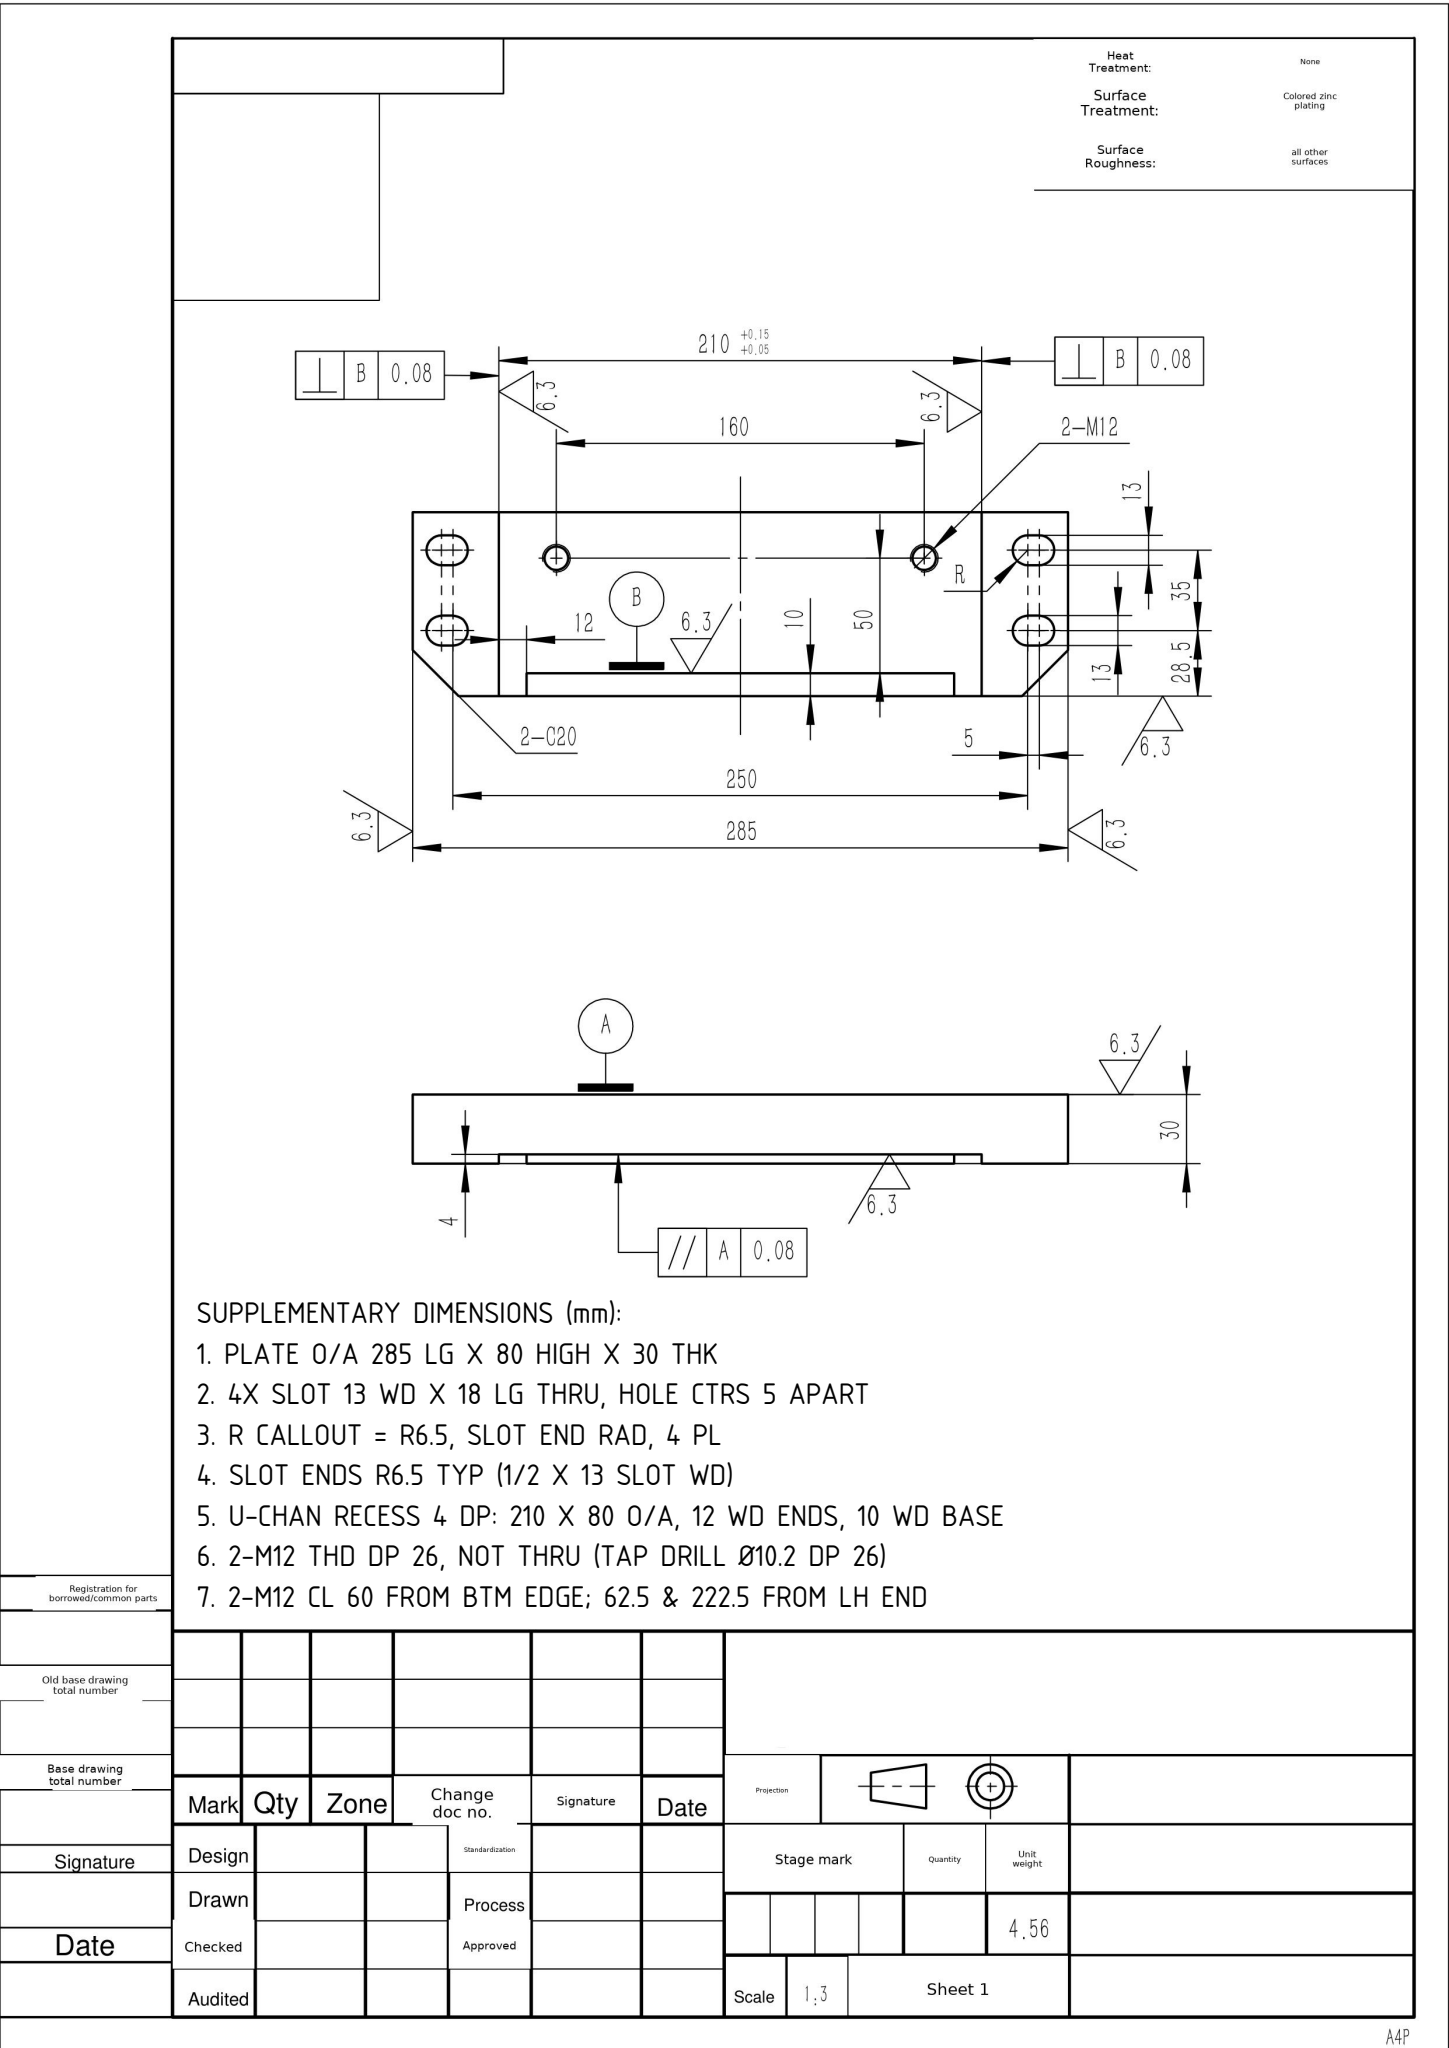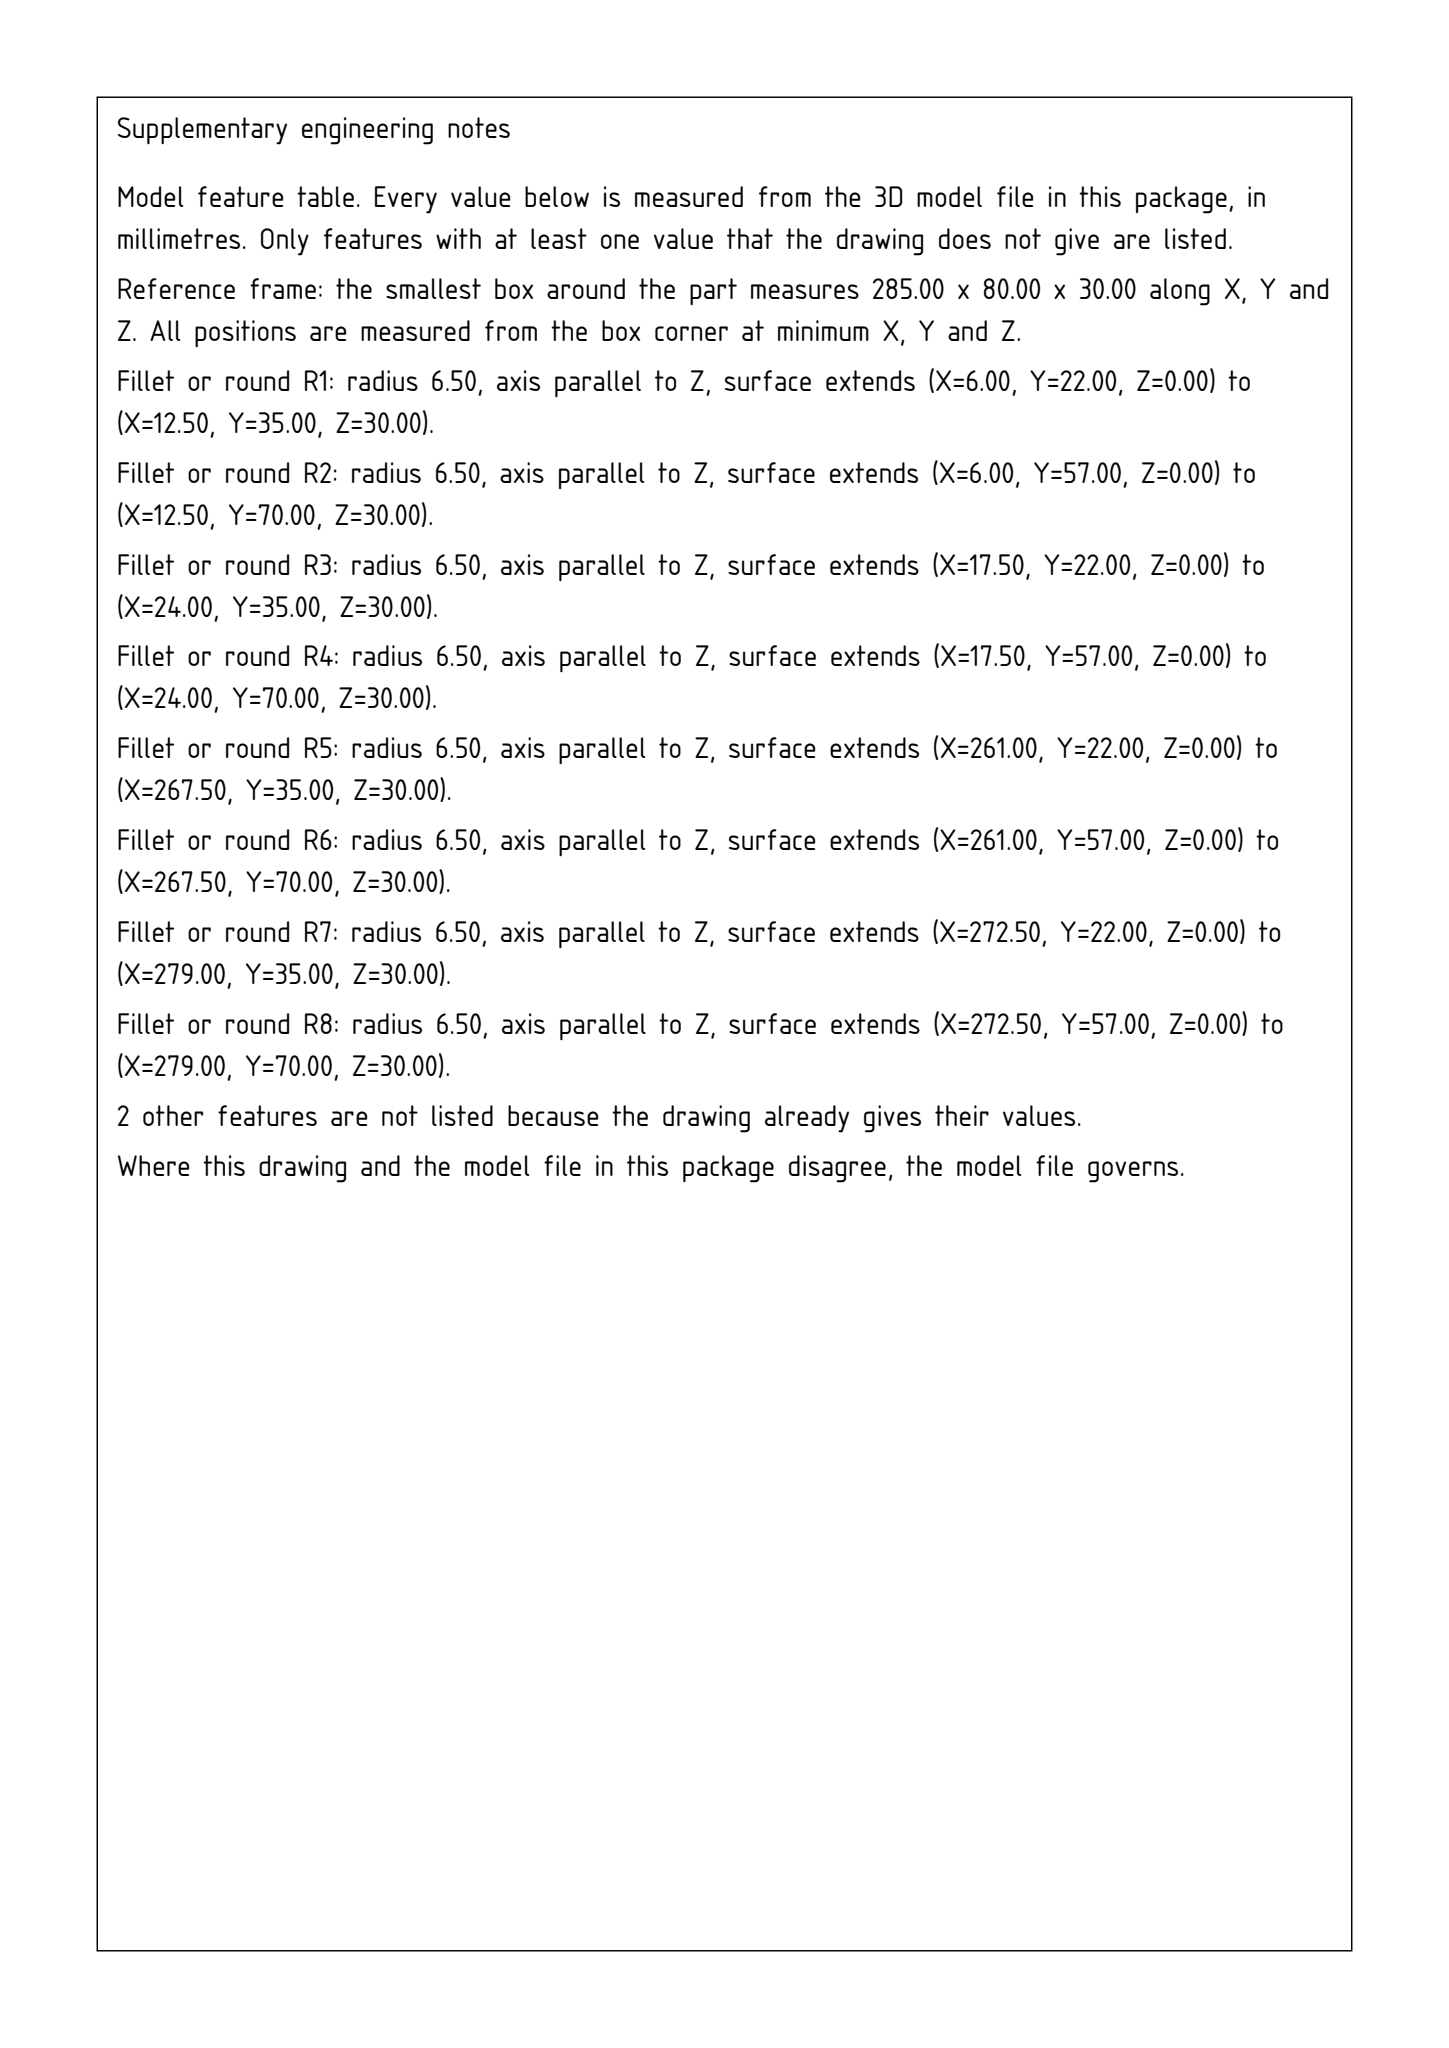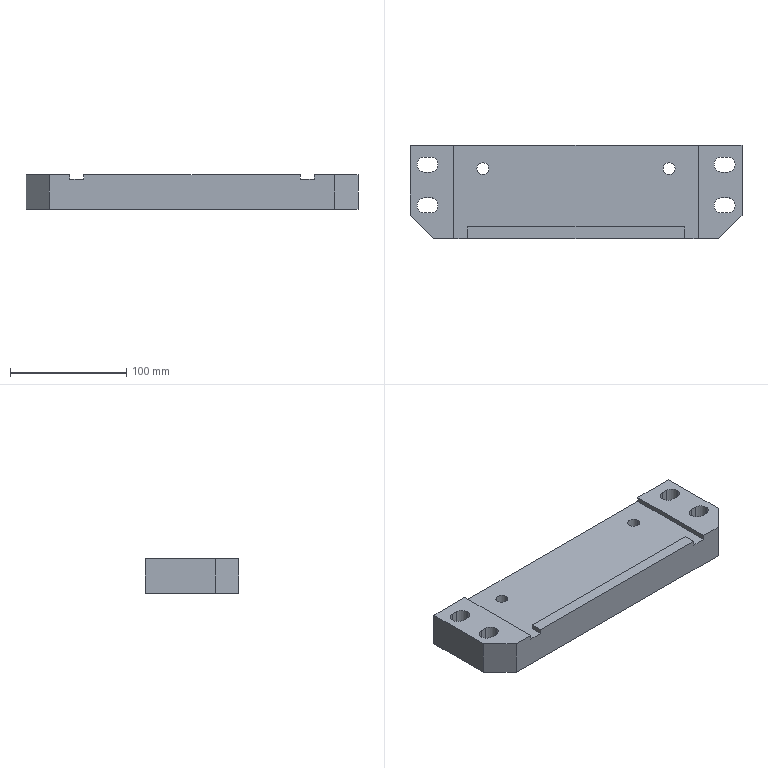Part | SolidWorks | mm | 1 solid | 40 faces | box 285 x 80 x 30 mm | volume 584263 mm3 | plane 24 | cylinder 16 | commonest cylinder face diameters 13 x12 10.2 x4
build123d program:
from build123d import *

# Parameters (mm, degrees)
SKETCH1_W              = 285
SKETCH1_H              = 80
BOSS_EXTRUDE1_DEPTH    = 30
CUT_EXTRUDE1_DEPTH     = 4
CUT_EXTRUDE2_DEPTH     = 152.017
CHAMFER1_SIZE          = 20
M12_TAPPED_HOLE1_D     = 10.2
M12_TAPPED_HOLE1_DEPTH = 29.25
M12_TAPPED_HOLE1_TIP   = 3.064


with BuildPart() as part:
    # Sketch1 → Boss-Extrude1 (new body)
    with BuildSketch(Plane.XY):
        Rectangle(SKETCH1_W, SKETCH1_H)
    extrude(amount=BOSS_EXTRUDE1_DEPTH)

    # Sketch2 → Cut-Extrude1 (cut)
    with BuildSketch(Plane.XY.offset(30)):
        Polygon((-105, 40), (105, 40), (105, -40), (93, -40), (93, -30), (-93, -30), (-93, -40), (-105, -40), align=None)
    extrude(amount=-CUT_EXTRUDE1_DEPTH, mode=Mode.SUBTRACT)

    # Sketch3 → Cut-Extrude2 (cut, through all)
    with BuildSketch(Plane.XY.offset(30)):
        with BuildLine():
            Line((-130, 30), (-125, 30))
            ThreePointArc((-125, 30), (-118.5, 23.5), (-125, 17))
            Line((-125, 17), (-130, 17))
            ThreePointArc((-130, 17), (-136.5, 23.5), (-130, 30))
        make_face()
        with BuildLine():
            Line((130, 30), (125, 30))
            ThreePointArc((125, 30), (118.5, 23.5), (125, 17))
            Line((125, 17), (130, 17))
            ThreePointArc((130, 17), (136.5, 23.5), (130, 30))
        make_face()
        with BuildLine():
            Line((-130, -5), (-125, -5))
            ThreePointArc((-125, -5), (-118.5, -11.5), (-125, -18))
            Line((-125, -18), (-130, -18))
            ThreePointArc((-130, -18), (-136.5, -11.5), (-130, -5))
        make_face()
        with BuildLine():
            Line((130, -5), (125, -5))
            ThreePointArc((125, -5), (118.5, -11.5), (125, -18))
            Line((125, -18), (130, -18))
            ThreePointArc((130, -18), (136.5, -11.5), (130, -5))
        make_face()
    extrude(amount=-CUT_EXTRUDE2_DEPTH, mode=Mode.SUBTRACT)

    # Chamfer1
    chamfer1_edges = [part.edges().sort_by_distance(p)[0] for p in [
        (142.5, -40, 15),
        (-142.5, -40, 15),
    ]]
    chamfer(chamfer1_edges, length=CHAMFER1_SIZE)

    # M12 Tapped Hole1
    with Locations(Plane.XY.offset(26)):
        with Locations((-80, 20), (80, 20)):
            Hole(M12_TAPPED_HOLE1_D / 2, depth=M12_TAPPED_HOLE1_DEPTH)
            with Locations((0, 0, -(M12_TAPPED_HOLE1_DEPTH + M12_TAPPED_HOLE1_TIP / 2))):  # 118° drill point
                Cone(0, M12_TAPPED_HOLE1_D / 2, M12_TAPPED_HOLE1_TIP, mode=Mode.SUBTRACT)


solid = part.part